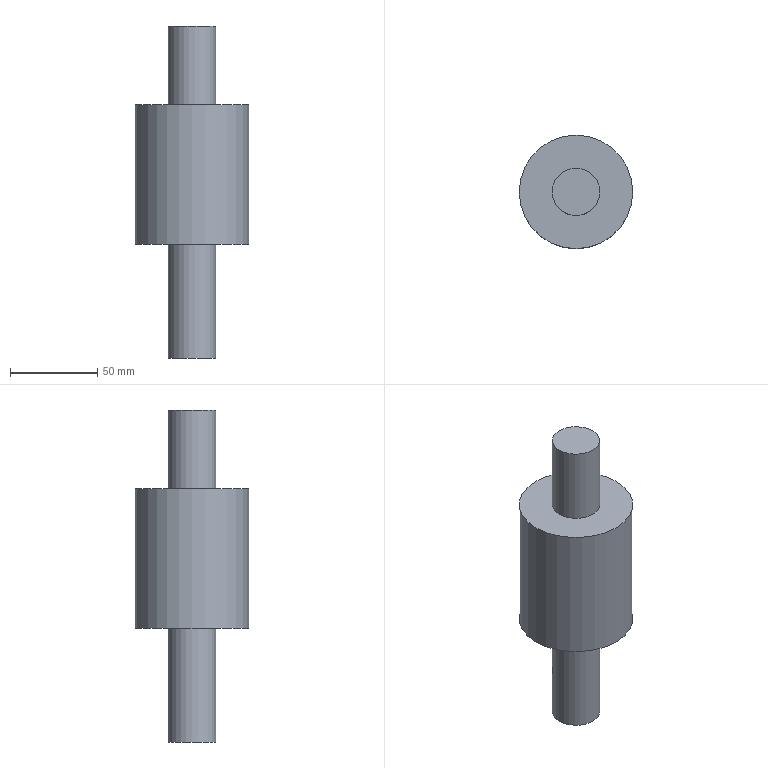Component | NX | LOCATING_PIN | 1 solid | 7 faces | box 65 x 65 x 190 mm | volume 329187 mm3 | plane 4 | cylinder 3 | commonest cylinder face diameters 27.158 x2 65 x1
STEP:
#1=CARTESIAN_POINT('',(0.,0.,0.));
#2=DIRECTION('',(0.,0.,1.));
#3=DIRECTION('',(1.,0.,0.));
#4=AXIS2_PLACEMENT_3D('',#1,#2,#3);
#5=CARTESIAN_POINT('',(32.5,0.,113.));
#6=VERTEX_POINT('',#5);
#7=CARTESIAN_POINT('',(-0.,0.,113.));
#8=DIRECTION('',(0.,0.,1.));
#9=DIRECTION('',(1.,0.,0.));
#10=AXIS2_PLACEMENT_3D('',#7,#8,#9);
#11=CIRCLE('',#10,32.5);
#12=CARTESIAN_POINT('',(-0.,0.,113.));
#13=DIRECTION('',(0.,0.,-1.));
#14=DIRECTION('',(-1.,0.,0.));
#15=AXIS2_PLACEMENT_3D('',#12,#13,#14);
#16=CYLINDRICAL_SURFACE('',#15,32.5);
#17=CARTESIAN_POINT('',(9.425,0.));
#18=DIRECTION('',(-1.,0.));
#19=VECTOR('',#18,1.);
#20=LINE('',#17,#19);
#21=(GEOMETRIC_REPRESENTATION_CONTEXT(2)PARAMETRIC_REPRESENTATION_CONTEXT()REPRESENTATION_CONTEXT('',''));
#22=DEFINITIONAL_REPRESENTATION('',(#20),#21);
#23=PCURVE('',#16,#22);
#24=CARTESIAN_POINT('',(-0.,0.,113.));
#25=DIRECTION('',(0.,0.,1.));
#26=DIRECTION('',(1.,0.,0.));
#27=AXIS2_PLACEMENT_3D('',#24,#25,#26);
#28=PLANE('',#27);
#29=CARTESIAN_POINT('',(0.,0.));
#30=DIRECTION('',(1.,0.));
#31=AXIS2_PLACEMENT_2D('',#29,#30);
#32=CIRCLE('',#31,32.5);
#33=(GEOMETRIC_REPRESENTATION_CONTEXT(2)PARAMETRIC_REPRESENTATION_CONTEXT()REPRESENTATION_CONTEXT('',''));
#34=DEFINITIONAL_REPRESENTATION('',(#32),#33);
#35=PCURVE('',#28,#34);
#36=SURFACE_CURVE('',#11,(#23,#35),.PCURVE_S1.);
#37=EDGE_CURVE('',#6,#6,#36,.T.);
#38=ORIENTED_EDGE('',*,*,#37,.F.);
#39=CARTESIAN_POINT('',(32.5,0.,33.));
#40=VERTEX_POINT('',#39);
#41=CARTESIAN_POINT('',(32.5,0.,113.));
#42=CARTESIAN_POINT('',(32.5,0.,33.));
#43=B_SPLINE_CURVE_WITH_KNOTS('',1,(#41,#42),.UNSPECIFIED.,.F.,.F.,(2,2),(0.,80.),.PIECEWISE_BEZIER_KNOTS.);
#44=CARTESIAN_POINT('',(9.425,0.));
#45=DIRECTION('',(0.,1.));
#46=VECTOR('',#45,1.);
#47=LINE('',#44,#46);
#48=(GEOMETRIC_REPRESENTATION_CONTEXT(2)PARAMETRIC_REPRESENTATION_CONTEXT()REPRESENTATION_CONTEXT('',''));
#49=DEFINITIONAL_REPRESENTATION('',(#47),#48);
#50=PCURVE('',#16,#49);
#51=CARTESIAN_POINT('',(3.142,0.));
#52=DIRECTION('',(0.,1.));
#53=VECTOR('',#52,1.);
#54=LINE('',#51,#53);
#55=(GEOMETRIC_REPRESENTATION_CONTEXT(2)PARAMETRIC_REPRESENTATION_CONTEXT()REPRESENTATION_CONTEXT('',''));
#56=DEFINITIONAL_REPRESENTATION('',(#54),#55);
#57=PCURVE('',#16,#56);
#58=SEAM_CURVE('',#43,(#50,#57),.PCURVE_S1.);
#59=EDGE_CURVE('',#6,#40,#58,.T.);
#60=ORIENTED_EDGE('',*,*,#59,.T.);
#61=CARTESIAN_POINT('',(-0.,0.,33.));
#62=DIRECTION('',(0.,0.,1.));
#63=DIRECTION('',(1.,0.,0.));
#64=AXIS2_PLACEMENT_3D('',#61,#62,#63);
#65=CIRCLE('',#64,32.5);
#66=CARTESIAN_POINT('',(9.425,80.));
#67=DIRECTION('',(-1.,0.));
#68=VECTOR('',#67,1.);
#69=LINE('',#66,#68);
#70=(GEOMETRIC_REPRESENTATION_CONTEXT(2)PARAMETRIC_REPRESENTATION_CONTEXT()REPRESENTATION_CONTEXT('',''));
#71=DEFINITIONAL_REPRESENTATION('',(#69),#70);
#72=PCURVE('',#16,#71);
#73=CARTESIAN_POINT('',(-0.,0.,33.));
#74=DIRECTION('',(0.,0.,1.));
#75=DIRECTION('',(1.,0.,0.));
#76=AXIS2_PLACEMENT_3D('',#73,#74,#75);
#77=PLANE('',#76);
#78=CARTESIAN_POINT('',(0.,0.));
#79=DIRECTION('',(1.,0.));
#80=AXIS2_PLACEMENT_2D('',#78,#79);
#81=CIRCLE('',#80,32.5);
#82=(GEOMETRIC_REPRESENTATION_CONTEXT(2)PARAMETRIC_REPRESENTATION_CONTEXT()REPRESENTATION_CONTEXT('',''));
#83=DEFINITIONAL_REPRESENTATION('',(#81),#82);
#84=PCURVE('',#77,#83);
#85=SURFACE_CURVE('',#65,(#72,#84),.PCURVE_S1.);
#86=EDGE_CURVE('',#40,#40,#85,.T.);
#87=ORIENTED_EDGE('',*,*,#86,.T.);
#88=ORIENTED_EDGE('',*,*,#59,.F.);
#89=EDGE_LOOP('',(#38,#60,#87,#88));
#90=FACE_BOUND('',#89,.T.);
#91=ADVANCED_FACE('',(#90),#16,.T.);
#92=CARTESIAN_POINT('',(13.579,0.,113.));
#93=VERTEX_POINT('',#92);
#94=CARTESIAN_POINT('',(-0.,0.,113.));
#95=DIRECTION('',(0.,0.,1.));
#96=DIRECTION('',(1.,0.,0.));
#97=AXIS2_PLACEMENT_3D('',#94,#95,#96);
#98=CIRCLE('',#97,13.579);
#99=CARTESIAN_POINT('',(0.,0.));
#100=DIRECTION('',(1.,0.));
#101=AXIS2_PLACEMENT_2D('',#99,#100);
#102=CIRCLE('',#101,13.579);
#103=(GEOMETRIC_REPRESENTATION_CONTEXT(2)PARAMETRIC_REPRESENTATION_CONTEXT()REPRESENTATION_CONTEXT('',''));
#104=DEFINITIONAL_REPRESENTATION('',(#102),#103);
#105=PCURVE('',#28,#104);
#106=CARTESIAN_POINT('',(-0.,0.,158.));
#107=DIRECTION('',(0.,0.,-1.));
#108=DIRECTION('',(-1.,0.,0.));
#109=AXIS2_PLACEMENT_3D('',#106,#107,#108);
#110=CYLINDRICAL_SURFACE('',#109,13.579);
#111=CARTESIAN_POINT('',(9.425,45.));
#112=DIRECTION('',(-1.,0.));
#113=VECTOR('',#112,1.);
#114=LINE('',#111,#113);
#115=(GEOMETRIC_REPRESENTATION_CONTEXT(2)PARAMETRIC_REPRESENTATION_CONTEXT()REPRESENTATION_CONTEXT('',''));
#116=DEFINITIONAL_REPRESENTATION('',(#114),#115);
#117=PCURVE('',#110,#116);
#118=SURFACE_CURVE('',#98,(#105,#117),.PCURVE_S1.);
#119=EDGE_CURVE('',#93,#93,#118,.T.);
#120=ORIENTED_EDGE('',*,*,#119,.F.);
#121=EDGE_LOOP('',(#120));
#122=FACE_BOUND('',#121,.T.);
#123=ORIENTED_EDGE('',*,*,#37,.T.);
#124=EDGE_LOOP('',(#123));
#125=FACE_BOUND('',#124,.T.);
#126=ADVANCED_FACE('',(#122,#125),#28,.T.);
#127=CARTESIAN_POINT('',(13.579,0.,33.));
#128=VERTEX_POINT('',#127);
#129=CARTESIAN_POINT('',(-0.,0.,33.));
#130=DIRECTION('',(0.,0.,-1.));
#131=DIRECTION('',(1.,0.,0.));
#132=AXIS2_PLACEMENT_3D('',#129,#130,#131);
#133=CIRCLE('',#132,13.579);
#134=CARTESIAN_POINT('',(13.579,0.));
#135=CARTESIAN_POINT('',(13.579,-23.52));
#136=CARTESIAN_POINT('',(-6.79,-11.76));
#137=CARTESIAN_POINT('',(-27.158,-0.));
#138=CARTESIAN_POINT('',(-6.79,11.76));
#139=CARTESIAN_POINT('',(13.579,23.52));
#140=CARTESIAN_POINT('',(13.579,0.));
#141=(BOUNDED_CURVE()B_SPLINE_CURVE(2,(#134,#135,#136,#137,#138,#139,#140),.UNSPECIFIED.,.T.,.F.)B_SPLINE_CURVE_WITH_KNOTS((1,2,2,2,2,1),(-2.094,0.,2.094,4.189,6.283,8.378),.UNSPECIFIED.)CURVE()GEOMETRIC_REPRESENTATION_ITEM()RATIONAL_B_SPLINE_CURVE((1.,0.5,1.,0.5,1.,0.5,1.))REPRESENTATION_ITEM(''));
#142=(GEOMETRIC_REPRESENTATION_CONTEXT(2)PARAMETRIC_REPRESENTATION_CONTEXT()REPRESENTATION_CONTEXT('',''));
#143=DEFINITIONAL_REPRESENTATION('',(#141),#142);
#144=PCURVE('',#77,#143);
#145=CARTESIAN_POINT('',(-0.,0.,-32.));
#146=DIRECTION('',(0.,0.,1.));
#147=DIRECTION('',(1.,0.,0.));
#148=AXIS2_PLACEMENT_3D('',#145,#146,#147);
#149=CYLINDRICAL_SURFACE('',#148,13.579);
#150=CARTESIAN_POINT('',(6.283,65.));
#151=DIRECTION('',(-1.,0.));
#152=VECTOR('',#151,1.);
#153=LINE('',#150,#152);
#154=(GEOMETRIC_REPRESENTATION_CONTEXT(2)PARAMETRIC_REPRESENTATION_CONTEXT()REPRESENTATION_CONTEXT('',''));
#155=DEFINITIONAL_REPRESENTATION('',(#153),#154);
#156=PCURVE('',#149,#155);
#157=SURFACE_CURVE('',#133,(#144,#156),.PCURVE_S1.);
#158=EDGE_CURVE('',#128,#128,#157,.T.);
#159=ORIENTED_EDGE('',*,*,#158,.F.);
#160=EDGE_LOOP('',(#159));
#161=FACE_BOUND('',#160,.T.);
#162=ORIENTED_EDGE('',*,*,#86,.F.);
#163=EDGE_LOOP('',(#162));
#164=FACE_BOUND('',#163,.T.);
#165=ADVANCED_FACE('',(#161,#164),#77,.F.);
#166=CARTESIAN_POINT('',(13.579,0.,158.));
#167=VERTEX_POINT('',#166);
#168=CARTESIAN_POINT('',(-0.,0.,158.));
#169=DIRECTION('',(0.,0.,1.));
#170=DIRECTION('',(1.,0.,0.));
#171=AXIS2_PLACEMENT_3D('',#168,#169,#170);
#172=CIRCLE('',#171,13.579);
#173=CARTESIAN_POINT('',(9.425,0.));
#174=DIRECTION('',(-1.,0.));
#175=VECTOR('',#174,1.);
#176=LINE('',#173,#175);
#177=(GEOMETRIC_REPRESENTATION_CONTEXT(2)PARAMETRIC_REPRESENTATION_CONTEXT()REPRESENTATION_CONTEXT('',''));
#178=DEFINITIONAL_REPRESENTATION('',(#176),#177);
#179=PCURVE('',#110,#178);
#180=CARTESIAN_POINT('',(-0.,0.,158.));
#181=DIRECTION('',(0.,0.,1.));
#182=DIRECTION('',(1.,0.,0.));
#183=AXIS2_PLACEMENT_3D('',#180,#181,#182);
#184=PLANE('',#183);
#185=CARTESIAN_POINT('',(0.,0.));
#186=DIRECTION('',(1.,0.));
#187=AXIS2_PLACEMENT_2D('',#185,#186);
#188=CIRCLE('',#187,13.579);
#189=(GEOMETRIC_REPRESENTATION_CONTEXT(2)PARAMETRIC_REPRESENTATION_CONTEXT()REPRESENTATION_CONTEXT('',''));
#190=DEFINITIONAL_REPRESENTATION('',(#188),#189);
#191=PCURVE('',#184,#190);
#192=SURFACE_CURVE('',#172,(#179,#191),.PCURVE_S1.);
#193=EDGE_CURVE('',#167,#167,#192,.T.);
#194=ORIENTED_EDGE('',*,*,#193,.F.);
#195=CARTESIAN_POINT('',(13.579,0.,158.));
#196=CARTESIAN_POINT('',(13.579,0.,113.));
#197=B_SPLINE_CURVE_WITH_KNOTS('',1,(#195,#196),.UNSPECIFIED.,.F.,.F.,(2,2),(0.,45.),.PIECEWISE_BEZIER_KNOTS.);
#198=CARTESIAN_POINT('',(9.425,0.));
#199=DIRECTION('',(0.,1.));
#200=VECTOR('',#199,1.);
#201=LINE('',#198,#200);
#202=(GEOMETRIC_REPRESENTATION_CONTEXT(2)PARAMETRIC_REPRESENTATION_CONTEXT()REPRESENTATION_CONTEXT('',''));
#203=DEFINITIONAL_REPRESENTATION('',(#201),#202);
#204=PCURVE('',#110,#203);
#205=CARTESIAN_POINT('',(3.142,0.));
#206=DIRECTION('',(0.,1.));
#207=VECTOR('',#206,1.);
#208=LINE('',#205,#207);
#209=(GEOMETRIC_REPRESENTATION_CONTEXT(2)PARAMETRIC_REPRESENTATION_CONTEXT()REPRESENTATION_CONTEXT('',''));
#210=DEFINITIONAL_REPRESENTATION('',(#208),#209);
#211=PCURVE('',#110,#210);
#212=SEAM_CURVE('',#197,(#204,#211),.PCURVE_S1.);
#213=EDGE_CURVE('',#167,#93,#212,.T.);
#214=ORIENTED_EDGE('',*,*,#213,.T.);
#215=ORIENTED_EDGE('',*,*,#119,.T.);
#216=ORIENTED_EDGE('',*,*,#213,.F.);
#217=EDGE_LOOP('',(#194,#214,#215,#216));
#218=FACE_BOUND('',#217,.T.);
#219=ADVANCED_FACE('',(#218),#110,.T.);
#220=ORIENTED_EDGE('',*,*,#193,.T.);
#221=EDGE_LOOP('',(#220));
#222=FACE_BOUND('',#221,.T.);
#223=ADVANCED_FACE('',(#222),#184,.T.);
#224=CARTESIAN_POINT('',(13.579,0.,-32.));
#225=VERTEX_POINT('',#224);
#226=CARTESIAN_POINT('',(-0.,0.,-32.));
#227=DIRECTION('',(0.,0.,-1.));
#228=DIRECTION('',(1.,0.,0.));
#229=AXIS2_PLACEMENT_3D('',#226,#227,#228);
#230=CIRCLE('',#229,13.579);
#231=CARTESIAN_POINT('',(6.283,0.));
#232=DIRECTION('',(-1.,0.));
#233=VECTOR('',#232,1.);
#234=LINE('',#231,#233);
#235=(GEOMETRIC_REPRESENTATION_CONTEXT(2)PARAMETRIC_REPRESENTATION_CONTEXT()REPRESENTATION_CONTEXT('',''));
#236=DEFINITIONAL_REPRESENTATION('',(#234),#235);
#237=PCURVE('',#149,#236);
#238=CARTESIAN_POINT('',(-0.,0.,-32.));
#239=DIRECTION('',(0.,0.,-1.));
#240=DIRECTION('',(-1.,0.,0.));
#241=AXIS2_PLACEMENT_3D('',#238,#239,#240);
#242=PLANE('',#241);
#243=CARTESIAN_POINT('',(0.,0.));
#244=DIRECTION('',(-1.,0.));
#245=AXIS2_PLACEMENT_2D('',#243,#244);
#246=CIRCLE('',#245,13.579);
#247=(GEOMETRIC_REPRESENTATION_CONTEXT(2)PARAMETRIC_REPRESENTATION_CONTEXT()REPRESENTATION_CONTEXT('',''));
#248=DEFINITIONAL_REPRESENTATION('',(#246),#247);
#249=PCURVE('',#242,#248);
#250=SURFACE_CURVE('',#230,(#237,#249),.PCURVE_S1.);
#251=EDGE_CURVE('',#225,#225,#250,.T.);
#252=ORIENTED_EDGE('',*,*,#251,.F.);
#253=CARTESIAN_POINT('',(13.579,0.,-32.));
#254=CARTESIAN_POINT('',(13.579,0.,33.));
#255=B_SPLINE_CURVE_WITH_KNOTS('',1,(#253,#254),.UNSPECIFIED.,.F.,.F.,(2,2),(0.,65.),.PIECEWISE_BEZIER_KNOTS.);
#256=CARTESIAN_POINT('',(6.283,0.));
#257=DIRECTION('',(0.,1.));
#258=VECTOR('',#257,1.);
#259=LINE('',#256,#258);
#260=(GEOMETRIC_REPRESENTATION_CONTEXT(2)PARAMETRIC_REPRESENTATION_CONTEXT()REPRESENTATION_CONTEXT('',''));
#261=DEFINITIONAL_REPRESENTATION('',(#259),#260);
#262=PCURVE('',#149,#261);
#263=CARTESIAN_POINT('',(0.,0.));
#264=DIRECTION('',(0.,1.));
#265=VECTOR('',#264,1.);
#266=LINE('',#263,#265);
#267=(GEOMETRIC_REPRESENTATION_CONTEXT(2)PARAMETRIC_REPRESENTATION_CONTEXT()REPRESENTATION_CONTEXT('',''));
#268=DEFINITIONAL_REPRESENTATION('',(#266),#267);
#269=PCURVE('',#149,#268);
#270=SEAM_CURVE('',#255,(#262,#269),.PCURVE_S1.);
#271=EDGE_CURVE('',#225,#128,#270,.T.);
#272=ORIENTED_EDGE('',*,*,#271,.T.);
#273=ORIENTED_EDGE('',*,*,#158,.T.);
#274=ORIENTED_EDGE('',*,*,#271,.F.);
#275=EDGE_LOOP('',(#252,#272,#273,#274));
#276=FACE_BOUND('',#275,.T.);
#277=ADVANCED_FACE('',(#276),#149,.T.);
#278=ORIENTED_EDGE('',*,*,#251,.T.);
#279=EDGE_LOOP('',(#278));
#280=FACE_BOUND('',#279,.T.);
#281=ADVANCED_FACE('',(#280),#242,.T.);
#282=CLOSED_SHELL('',(#91,#126,#165,#219,#223,#277,#281));
#283=MANIFOLD_SOLID_BREP('',#282);
#284=(LENGTH_UNIT()NAMED_UNIT(*)SI_UNIT(.MILLI.,.METRE.));
#285=UNCERTAINTY_MEASURE_WITH_UNIT(LENGTH_MEASURE(0.00001),#284,'','');
#286=(NAMED_UNIT(*)PLANE_ANGLE_UNIT()SI_UNIT($,.RADIAN.));
#287=(NAMED_UNIT(*)SI_UNIT($,.STERADIAN.)SOLID_ANGLE_UNIT());
#288=(GEOMETRIC_REPRESENTATION_CONTEXT(3)GLOBAL_UNCERTAINTY_ASSIGNED_CONTEXT((#285))GLOBAL_UNIT_ASSIGNED_CONTEXT((#284,#286,#287))REPRESENTATION_CONTEXT('',''));
#289=ADVANCED_BREP_SHAPE_REPRESENTATION('',(#4,#283),#288);